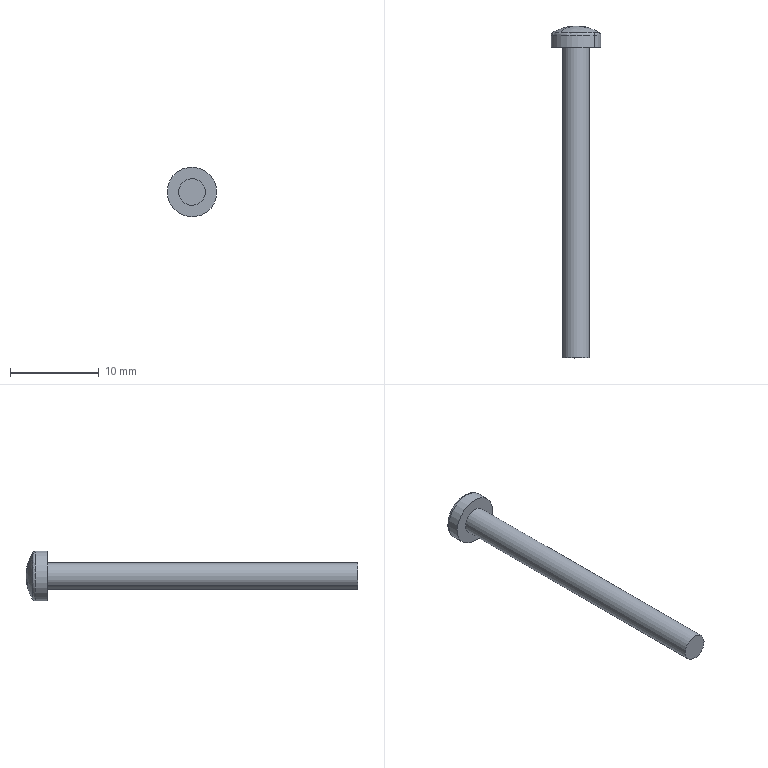Component | SolidWorks | pan cross head_am_pkg-12 | 1 solid | 23 faces | box 5.6 x 37.39 x 5.6 mm | volume 294 mm3 | plane 15 | cylinder 4 | torus 2 | sphere 2 | commonest cylinder face diameters 5.6 x2 3 x2
STEP:
#1=COLOUR_RGB('',0.7922,0.8196,0.9333);
#2=FILL_AREA_STYLE_COLOUR('',#1);
#3=FILL_AREA_STYLE('',(#2));
#4=SURFACE_STYLE_FILL_AREA(#3);
#5=SURFACE_SIDE_STYLE('',(#4));
#6=SURFACE_STYLE_USAGE(.BOTH.,#5);
#7=PRESENTATION_STYLE_ASSIGNMENT((#6));
#8=CARTESIAN_POINT('',(-1.144,1.16,0.966));
#9=VERTEX_POINT('',#8);
#10=CARTESIAN_POINT('',(-1.306,1.16,0.8157));
#11=VERTEX_POINT('',#10);
#12=CARTESIAN_POINT('',(-1.225,1.16,0.8908));
#13=DIRECTION('',(-0.,1.,-0.));
#14=DIRECTION('',(0.7319,0.,0.6814));
#15=AXIS2_PLACEMENT_3D('',#12,#13,#14);
#16=CIRCLE('',#15,0.1102);
#17=EDGE_CURVE('',#9,#11,#16,.T.);
#18=ORIENTED_EDGE('',*,*,#17,.T.);
#19=CARTESIAN_POINT('',(-1.301,1.171,0.82));
#20=VERTEX_POINT('',#19);
#21=CARTESIAN_POINT('',(-1.296,1.16,0.8247));
#22=DIRECTION('',(0.6814,0.,-0.7319));
#23=DIRECTION('',(-0.7319,0.,-0.6814));
#24=AXIS2_PLACEMENT_3D('',#21,#22,#23);
#25=CIRCLE('',#24,0.01323);
#26=EDGE_CURVE('',#11,#20,#25,.T.);
#27=ORIENTED_EDGE('',*,*,#26,.T.);
#28=CARTESIAN_POINT('',(-1.154,1.171,0.8147));
#29=VERTEX_POINT('',#28);
#30=CARTESIAN_POINT('',(-1.225,1.171,0.8908));
#31=DIRECTION('',(-0.,1.,-0.));
#32=DIRECTION('',(0.7319,0.,0.6814));
#33=AXIS2_PLACEMENT_3D('',#30,#31,#32);
#34=CIRCLE('',#33,0.104);
#35=EDGE_CURVE('',#29,#20,#34,.T.);
#36=ORIENTED_EDGE('',*,*,#35,.F.);
#37=CARTESIAN_POINT('',(-1.149,1.171,0.9617));
#38=VERTEX_POINT('',#37);
#39=CARTESIAN_POINT('',(-1.225,1.171,0.8908));
#40=DIRECTION('',(-0.,1.,-0.));
#41=DIRECTION('',(0.7319,0.,0.6814));
#42=AXIS2_PLACEMENT_3D('',#39,#40,#41);
#43=CIRCLE('',#42,0.104);
#44=EDGE_CURVE('',#38,#29,#43,.T.);
#45=ORIENTED_EDGE('',*,*,#44,.F.);
#46=CARTESIAN_POINT('',(-1.154,1.16,0.9569));
#47=DIRECTION('',(-0.6814,-0.,0.7319));
#48=DIRECTION('',(0.7319,0.,0.6814));
#49=AXIS2_PLACEMENT_3D('',#46,#47,#48);
#50=CIRCLE('',#49,0.01323);
#51=EDGE_CURVE('',#9,#38,#50,.T.);
#52=ORIENTED_EDGE('',*,*,#51,.F.);
#53=EDGE_LOOP('',(#18,#27,#36,#45,#52));
#54=FACE_OUTER_BOUND('',#53,.T.);
#55=CARTESIAN_POINT('',(-1.225,1.16,0.8908));
#56=DIRECTION('',(-0.,1.,-0.));
#57=DIRECTION('',(0.7319,0.,0.6814));
#58=AXIS2_PLACEMENT_3D('',#55,#56,#57);
#59=TOROIDAL_SURFACE('',#58,0.09701,0.01323);
#60=ADVANCED_FACE('',(#54),#59,.T.);
#61=CARTESIAN_POINT('',(-1.144,1.106,0.966));
#62=VERTEX_POINT('',#61);
#63=CARTESIAN_POINT('',(-1.306,1.106,0.8157));
#64=VERTEX_POINT('',#63);
#65=CARTESIAN_POINT('',(-1.225,1.106,0.8908));
#66=DIRECTION('',(-0.,1.,-0.));
#67=DIRECTION('',(0.7319,0.,0.6814));
#68=AXIS2_PLACEMENT_3D('',#65,#66,#67);
#69=CIRCLE('',#68,0.1102);
#70=EDGE_CURVE('',#62,#64,#69,.T.);
#71=ORIENTED_EDGE('',*,*,#70,.T.);
#72=CARTESIAN_POINT('',(-1.306,2.201,0.8157));
#73=DIRECTION('',(-0.,1.,-0.));
#74=VECTOR('',#73,39.37);
#75=LINE('',#72,#74);
#76=EDGE_CURVE('',#64,#11,#75,.T.);
#77=ORIENTED_EDGE('',*,*,#76,.T.);
#78=ORIENTED_EDGE('',*,*,#17,.F.);
#79=CARTESIAN_POINT('',(-1.144,2.201,0.966));
#80=DIRECTION('',(-0.,1.,-0.));
#81=VECTOR('',#80,39.37);
#82=LINE('',#79,#81);
#83=EDGE_CURVE('',#62,#9,#82,.T.);
#84=ORIENTED_EDGE('',*,*,#83,.F.);
#85=EDGE_LOOP('',(#71,#77,#78,#84));
#86=FACE_OUTER_BOUND('',#85,.T.);
#87=CARTESIAN_POINT('',(-1.225,2.201,0.8908));
#88=DIRECTION('',(-0.,1.,-0.));
#89=DIRECTION('',(0.7319,0.,0.6814));
#90=AXIS2_PLACEMENT_3D('',#87,#88,#89);
#91=CYLINDRICAL_SURFACE('',#90,0.1102);
#92=ADVANCED_FACE('',(#86),#91,.T.);
#93=CARTESIAN_POINT('',(-1.182,-0.2717,0.9311));
#94=VERTEX_POINT('',#93);
#95=CARTESIAN_POINT('',(-1.268,-0.2717,0.8506));
#96=VERTEX_POINT('',#95);
#97=CARTESIAN_POINT('',(-1.225,-0.2717,0.8908));
#98=DIRECTION('',(-0.,1.,-0.));
#99=DIRECTION('',(0.7319,0.,0.6814));
#100=AXIS2_PLACEMENT_3D('',#97,#98,#99);
#101=CIRCLE('',#100,0.05906);
#102=EDGE_CURVE('',#94,#96,#101,.T.);
#103=ORIENTED_EDGE('',*,*,#102,.T.);
#104=CARTESIAN_POINT('',(-1.268,1.106,0.8506));
#105=VERTEX_POINT('',#104);
#106=CARTESIAN_POINT('',(-1.268,2.201,0.8506));
#107=DIRECTION('',(-0.,1.,-0.));
#108=VECTOR('',#107,39.37);
#109=LINE('',#106,#108);
#110=EDGE_CURVE('',#96,#105,#109,.T.);
#111=ORIENTED_EDGE('',*,*,#110,.T.);
#112=CARTESIAN_POINT('',(-1.182,1.106,0.9311));
#113=VERTEX_POINT('',#112);
#114=CARTESIAN_POINT('',(-1.225,1.106,0.8908));
#115=DIRECTION('',(-0.,1.,-0.));
#116=DIRECTION('',(0.7319,0.,0.6814));
#117=AXIS2_PLACEMENT_3D('',#114,#115,#116);
#118=CIRCLE('',#117,0.05906);
#119=EDGE_CURVE('',#113,#105,#118,.T.);
#120=ORIENTED_EDGE('',*,*,#119,.F.);
#121=CARTESIAN_POINT('',(-1.182,2.201,0.9311));
#122=DIRECTION('',(-0.,1.,-0.));
#123=VECTOR('',#122,39.37);
#124=LINE('',#121,#123);
#125=EDGE_CURVE('',#94,#113,#124,.T.);
#126=ORIENTED_EDGE('',*,*,#125,.F.);
#127=EDGE_LOOP('',(#103,#111,#120,#126));
#128=FACE_OUTER_BOUND('',#127,.T.);
#129=CARTESIAN_POINT('',(-1.225,2.201,0.8908));
#130=DIRECTION('',(-0.,1.,-0.));
#131=DIRECTION('',(0.7319,0.,0.6814));
#132=AXIS2_PLACEMENT_3D('',#129,#130,#131);
#133=CYLINDRICAL_SURFACE('',#132,0.05906);
#134=ADVANCED_FACE('',(#128),#133,.T.);
#135=ORIENTED_EDGE('',*,*,#35,.T.);
#136=CARTESIAN_POINT('',(-1.296,1.171,0.967));
#137=VERTEX_POINT('',#136);
#138=CARTESIAN_POINT('',(-1.225,1.171,0.8908));
#139=DIRECTION('',(-0.,1.,-0.));
#140=DIRECTION('',(0.7319,0.,0.6814));
#141=AXIS2_PLACEMENT_3D('',#138,#139,#140);
#142=CIRCLE('',#141,0.104);
#143=EDGE_CURVE('',#20,#137,#142,.T.);
#144=ORIENTED_EDGE('',*,*,#143,.T.);
#145=CARTESIAN_POINT('',(-1.26,1.194,0.9286));
#146=VERTEX_POINT('',#145);
#147=CARTESIAN_POINT('',(-1.225,1.004,0.8908));
#148=DIRECTION('',(-0.7319,-0.,-0.6814));
#149=DIRECTION('',(-0.6814,0.,0.7319));
#150=AXIS2_PLACEMENT_3D('',#147,#148,#149);
#151=CIRCLE('',#150,0.1969);
#152=EDGE_CURVE('',#137,#146,#151,.T.);
#153=ORIENTED_EDGE('',*,*,#152,.T.);
#154=CARTESIAN_POINT('',(-1.267,1.194,0.9219));
#155=VERTEX_POINT('',#154);
#156=CARTESIAN_POINT('',(-1.19,1.038,0.8529));
#157=DIRECTION('',(-0.5674,-0.5538,0.6094));
#158=DIRECTION('',(0.3774,-0.8327,-0.4053));
#159=AXIS2_PLACEMENT_3D('',#156,#157,#158);
#160=CIRCLE('',#159,0.1867);
#161=EDGE_CURVE('',#146,#155,#160,.T.);
#162=ORIENTED_EDGE('',*,*,#161,.T.);
#163=CARTESIAN_POINT('',(-1.239,1.2,0.8914));
#164=VERTEX_POINT('',#163);
#165=CARTESIAN_POINT('',(-1.223,1.004,0.8928));
#166=DIRECTION('',(0.7303,0.06592,0.6799));
#167=DIRECTION('',(0.04824,-0.9978,0.04492));
#168=AXIS2_PLACEMENT_3D('',#165,#166,#167);
#169=CIRCLE('',#168,0.1968);
#170=EDGE_CURVE('',#164,#155,#169,.T.);
#171=ORIENTED_EDGE('',*,*,#170,.F.);
#172=CARTESIAN_POINT('',(-1.269,1.194,0.8629));
#173=VERTEX_POINT('',#172);
#174=CARTESIAN_POINT('',(-1.223,1.004,0.8888));
#175=DIRECTION('',(0.6799,0.06592,-0.7303));
#176=DIRECTION('',(-0.04492,0.9978,0.04824));
#177=AXIS2_PLACEMENT_3D('',#174,#175,#176);
#178=CIRCLE('',#177,0.1968);
#179=EDGE_CURVE('',#173,#164,#178,.T.);
#180=ORIENTED_EDGE('',*,*,#179,.F.);
#181=CARTESIAN_POINT('',(-1.256,1.194,0.8487));
#182=VERTEX_POINT('',#181);
#183=CARTESIAN_POINT('',(-1.187,1.038,0.9262));
#184=DIRECTION('',(-0.6094,-0.5538,-0.5674));
#185=DIRECTION('',(-0.4053,0.8327,-0.3774));
#186=AXIS2_PLACEMENT_3D('',#183,#184,#185);
#187=CIRCLE('',#186,0.1867);
#188=EDGE_CURVE('',#173,#182,#187,.T.);
#189=ORIENTED_EDGE('',*,*,#188,.T.);
#190=CARTESIAN_POINT('',(-1.225,1.2,0.8766));
#191=VERTEX_POINT('',#190);
#192=CARTESIAN_POINT('',(-1.227,1.004,0.8929));
#193=DIRECTION('',(-0.6799,0.06592,0.7303));
#194=DIRECTION('',(-0.04492,-0.9978,0.04824));
#195=AXIS2_PLACEMENT_3D('',#192,#193,#194);
#196=CIRCLE('',#195,0.1968);
#197=EDGE_CURVE('',#191,#182,#196,.T.);
#198=ORIENTED_EDGE('',*,*,#197,.F.);
#199=CARTESIAN_POINT('',(-1.197,1.194,0.8466));
#200=VERTEX_POINT('',#199);
#201=CARTESIAN_POINT('',(-1.223,1.004,0.8928));
#202=DIRECTION('',(0.7303,0.06592,0.6799));
#203=DIRECTION('',(0.04824,-0.9978,0.04492));
#204=AXIS2_PLACEMENT_3D('',#201,#202,#203);
#205=CIRCLE('',#204,0.1968);
#206=EDGE_CURVE('',#200,#191,#205,.T.);
#207=ORIENTED_EDGE('',*,*,#206,.F.);
#208=CARTESIAN_POINT('',(-1.19,1.194,0.8531));
#209=VERTEX_POINT('',#208);
#210=CARTESIAN_POINT('',(-1.26,1.038,0.9288));
#211=DIRECTION('',(0.5674,-0.5538,-0.6094));
#212=DIRECTION('',(0.3774,0.8327,-0.4053));
#213=AXIS2_PLACEMENT_3D('',#210,#211,#212);
#214=CIRCLE('',#213,0.1867);
#215=EDGE_CURVE('',#200,#209,#214,.T.);
#216=ORIENTED_EDGE('',*,*,#215,.T.);
#217=CARTESIAN_POINT('',(-1.225,1.004,0.8908));
#218=DIRECTION('',(0.7319,0.,0.6814));
#219=DIRECTION('',(0.6814,0.,-0.7319));
#220=AXIS2_PLACEMENT_3D('',#217,#218,#219);
#221=CIRCLE('',#220,0.1969);
#222=EDGE_CURVE('',#29,#209,#221,.T.);
#223=ORIENTED_EDGE('',*,*,#222,.F.);
#224=EDGE_LOOP('',(#135,#144,#153,#162,#171,#180,#189,#198,#207,#216,#223));
#225=FACE_OUTER_BOUND('',#224,.T.);
#226=CARTESIAN_POINT('',(-1.225,1.004,0.8908));
#227=DIRECTION('',(-0.7319,-0.,-0.6814));
#228=DIRECTION('',(0.6814,0.,-0.7319));
#229=AXIS2_PLACEMENT_3D('',#226,#227,#228);
#230=SPHERICAL_SURFACE('',#229,0.1969);
#231=ADVANCED_FACE('',(#225),#230,.T.);
#232=ORIENTED_EDGE('',*,*,#152,.F.);
#233=CARTESIAN_POINT('',(-1.225,1.171,0.8908));
#234=DIRECTION('',(-0.,1.,-0.));
#235=DIRECTION('',(0.7319,0.,0.6814));
#236=AXIS2_PLACEMENT_3D('',#233,#234,#235);
#237=CIRCLE('',#236,0.104);
#238=EDGE_CURVE('',#137,#38,#237,.T.);
#239=ORIENTED_EDGE('',*,*,#238,.T.);
#240=ORIENTED_EDGE('',*,*,#44,.T.);
#241=ORIENTED_EDGE('',*,*,#222,.T.);
#242=CARTESIAN_POINT('',(-1.183,1.194,0.8598));
#243=VERTEX_POINT('',#242);
#244=CARTESIAN_POINT('',(-1.26,1.038,0.9288));
#245=DIRECTION('',(0.5674,-0.5538,-0.6094));
#246=DIRECTION('',(0.3774,0.8327,-0.4053));
#247=AXIS2_PLACEMENT_3D('',#244,#245,#246);
#248=CIRCLE('',#247,0.1867);
#249=EDGE_CURVE('',#209,#243,#248,.T.);
#250=ORIENTED_EDGE('',*,*,#249,.T.);
#251=CARTESIAN_POINT('',(-1.211,1.2,0.8903));
#252=VERTEX_POINT('',#251);
#253=CARTESIAN_POINT('',(-1.227,1.004,0.8889));
#254=DIRECTION('',(-0.7303,0.06592,-0.6799));
#255=DIRECTION('',(0.04824,0.9978,0.04492));
#256=AXIS2_PLACEMENT_3D('',#253,#254,#255);
#257=CIRCLE('',#256,0.1968);
#258=EDGE_CURVE('',#252,#243,#257,.T.);
#259=ORIENTED_EDGE('',*,*,#258,.F.);
#260=CARTESIAN_POINT('',(-1.181,1.194,0.9188));
#261=VERTEX_POINT('',#260);
#262=CARTESIAN_POINT('',(-1.227,1.004,0.8929));
#263=DIRECTION('',(-0.6799,0.06592,0.7303));
#264=DIRECTION('',(-0.04492,-0.9978,0.04824));
#265=AXIS2_PLACEMENT_3D('',#262,#263,#264);
#266=CIRCLE('',#265,0.1968);
#267=EDGE_CURVE('',#261,#252,#266,.T.);
#268=ORIENTED_EDGE('',*,*,#267,.F.);
#269=CARTESIAN_POINT('',(-1.194,1.194,0.9329));
#270=VERTEX_POINT('',#269);
#271=CARTESIAN_POINT('',(-1.263,1.038,0.8555));
#272=DIRECTION('',(0.6094,-0.5538,0.5674));
#273=DIRECTION('',(-0.4053,-0.8327,-0.3774));
#274=AXIS2_PLACEMENT_3D('',#271,#272,#273);
#275=CIRCLE('',#274,0.1867);
#276=EDGE_CURVE('',#261,#270,#275,.T.);
#277=ORIENTED_EDGE('',*,*,#276,.T.);
#278=CARTESIAN_POINT('',(-1.224,1.2,0.9051));
#279=VERTEX_POINT('',#278);
#280=CARTESIAN_POINT('',(-1.223,1.004,0.8888));
#281=DIRECTION('',(0.6799,0.06592,-0.7303));
#282=DIRECTION('',(-0.04492,0.9978,0.04824));
#283=AXIS2_PLACEMENT_3D('',#280,#281,#282);
#284=CIRCLE('',#283,0.1968);
#285=EDGE_CURVE('',#279,#270,#284,.T.);
#286=ORIENTED_EDGE('',*,*,#285,.F.);
#287=CARTESIAN_POINT('',(-1.253,1.194,0.9351));
#288=VERTEX_POINT('',#287);
#289=CARTESIAN_POINT('',(-1.227,1.004,0.8889));
#290=DIRECTION('',(-0.7303,0.06592,-0.6799));
#291=DIRECTION('',(0.04824,0.9978,0.04492));
#292=AXIS2_PLACEMENT_3D('',#289,#290,#291);
#293=CIRCLE('',#292,0.1968);
#294=EDGE_CURVE('',#288,#279,#293,.T.);
#295=ORIENTED_EDGE('',*,*,#294,.F.);
#296=CARTESIAN_POINT('',(-1.19,1.038,0.8529));
#297=DIRECTION('',(-0.5674,-0.5538,0.6094));
#298=DIRECTION('',(0.3774,-0.8327,-0.4053));
#299=AXIS2_PLACEMENT_3D('',#296,#297,#298);
#300=CIRCLE('',#299,0.1867);
#301=EDGE_CURVE('',#288,#146,#300,.T.);
#302=ORIENTED_EDGE('',*,*,#301,.T.);
#303=EDGE_LOOP('',(#232,#239,#240,#241,#250,#259,#268,#277,#286,#295,#302));
#304=FACE_OUTER_BOUND('',#303,.T.);
#305=CARTESIAN_POINT('',(-1.225,1.004,0.8908));
#306=DIRECTION('',(-0.7319,-0.,-0.6814));
#307=DIRECTION('',(0.6814,0.,-0.7319));
#308=AXIS2_PLACEMENT_3D('',#305,#306,#307);
#309=SPHERICAL_SURFACE('',#308,0.1969);
#310=ADVANCED_FACE('',(#304),#309,.T.);
#311=ORIENTED_EDGE('',*,*,#206,.T.);
#312=CARTESIAN_POINT('',(-1.225,1.124,0.8837));
#313=VERTEX_POINT('',#312);
#314=CARTESIAN_POINT('',(-1.225,1.116,0.8844));
#315=DIRECTION('',(0.003322,-0.9957,0.09296));
#316=VECTOR('',#315,39.37);
#317=LINE('',#314,#316);
#318=EDGE_CURVE('',#191,#313,#317,.T.);
#319=ORIENTED_EDGE('',*,*,#318,.T.);
#320=CARTESIAN_POINT('',(-1.194,1.201,0.8429));
#321=DIRECTION('',(-0.3366,-0.8314,0.4421));
#322=VECTOR('',#321,39.37);
#323=LINE('',#320,#322);
#324=EDGE_CURVE('',#200,#313,#323,.T.);
#325=ORIENTED_EDGE('',*,*,#324,.F.);
#326=EDGE_LOOP('',(#311,#319,#325));
#327=FACE_OUTER_BOUND('',#326,.T.);
#328=CARTESIAN_POINT('',(-1.228,1.116,0.8877));
#329=DIRECTION('',(0.7303,0.06592,0.6799));
#330=DIRECTION('',(0.04824,-0.9978,0.04492));
#331=AXIS2_PLACEMENT_3D('',#328,#329,#330);
#332=PLANE('',#331);
#333=ADVANCED_FACE('',(#327),#332,.T.);
#334=CARTESIAN_POINT('',(-1.232,1.124,0.8911));
#335=VERTEX_POINT('',#334);
#336=CARTESIAN_POINT('',(-1.271,1.201,0.925));
#337=DIRECTION('',(0.417,-0.8314,-0.3673));
#338=VECTOR('',#337,39.37);
#339=LINE('',#336,#338);
#340=EDGE_CURVE('',#155,#335,#339,.T.);
#341=ORIENTED_EDGE('',*,*,#340,.T.);
#342=CARTESIAN_POINT('',(-1.231,1.116,0.8911));
#343=DIRECTION('',(-0.09296,0.9957,0.003322));
#344=VECTOR('',#343,39.37);
#345=LINE('',#342,#344);
#346=EDGE_CURVE('',#335,#164,#345,.T.);
#347=ORIENTED_EDGE('',*,*,#346,.T.);
#348=ORIENTED_EDGE('',*,*,#170,.T.);
#349=EDGE_LOOP('',(#341,#347,#348));
#350=FACE_OUTER_BOUND('',#349,.T.);
#351=CARTESIAN_POINT('',(-1.228,1.116,0.8877));
#352=DIRECTION('',(0.7303,0.06592,0.6799));
#353=DIRECTION('',(0.04824,-0.9978,0.04492));
#354=AXIS2_PLACEMENT_3D('',#351,#352,#353);
#355=PLANE('',#354);
#356=ADVANCED_FACE('',(#350),#355,.T.);
#357=CARTESIAN_POINT('',(-1.218,1.124,0.8906));
#358=VERTEX_POINT('',#357);
#359=CARTESIAN_POINT('',(-1.179,1.201,0.8567));
#360=DIRECTION('',(-0.417,-0.8314,0.3673));
#361=VECTOR('',#360,39.37);
#362=LINE('',#359,#361);
#363=EDGE_CURVE('',#243,#358,#362,.T.);
#364=ORIENTED_EDGE('',*,*,#363,.T.);
#365=CARTESIAN_POINT('',(-1.218,1.116,0.8906));
#366=DIRECTION('',(0.09296,0.9957,-0.003322));
#367=VECTOR('',#366,39.37);
#368=LINE('',#365,#367);
#369=EDGE_CURVE('',#358,#252,#368,.T.);
#370=ORIENTED_EDGE('',*,*,#369,.T.);
#371=ORIENTED_EDGE('',*,*,#258,.T.);
#372=EDGE_LOOP('',(#364,#370,#371));
#373=FACE_OUTER_BOUND('',#372,.T.);
#374=CARTESIAN_POINT('',(-1.222,1.116,0.894));
#375=DIRECTION('',(-0.7303,0.06592,-0.6799));
#376=DIRECTION('',(0.04824,0.9978,0.04492));
#377=AXIS2_PLACEMENT_3D('',#374,#375,#376);
#378=PLANE('',#377);
#379=ADVANCED_FACE('',(#373),#378,.T.);
#380=ORIENTED_EDGE('',*,*,#294,.T.);
#381=CARTESIAN_POINT('',(-1.225,1.124,0.898));
#382=VERTEX_POINT('',#381);
#383=CARTESIAN_POINT('',(-1.225,1.116,0.8973));
#384=DIRECTION('',(-0.003322,-0.9957,-0.09296));
#385=VECTOR('',#384,39.37);
#386=LINE('',#383,#385);
#387=EDGE_CURVE('',#279,#382,#386,.T.);
#388=ORIENTED_EDGE('',*,*,#387,.T.);
#389=CARTESIAN_POINT('',(-1.256,1.201,0.9388));
#390=DIRECTION('',(0.3366,-0.8314,-0.4421));
#391=VECTOR('',#390,39.37);
#392=LINE('',#389,#391);
#393=EDGE_CURVE('',#288,#382,#392,.T.);
#394=ORIENTED_EDGE('',*,*,#393,.F.);
#395=EDGE_LOOP('',(#380,#388,#394));
#396=FACE_OUTER_BOUND('',#395,.T.);
#397=CARTESIAN_POINT('',(-1.222,1.116,0.894));
#398=DIRECTION('',(-0.7303,0.06592,-0.6799));
#399=DIRECTION('',(0.04824,0.9978,0.04492));
#400=AXIS2_PLACEMENT_3D('',#397,#398,#399);
#401=PLANE('',#400);
#402=ADVANCED_FACE('',(#396),#401,.T.);
#403=ORIENTED_EDGE('',*,*,#110,.F.);
#404=CARTESIAN_POINT('',(-1.225,-0.2717,0.8908));
#405=DIRECTION('',(-0.,1.,-0.));
#406=DIRECTION('',(0.7319,0.,0.6814));
#407=AXIS2_PLACEMENT_3D('',#404,#405,#406);
#408=CIRCLE('',#407,0.05906);
#409=EDGE_CURVE('',#96,#94,#408,.T.);
#410=ORIENTED_EDGE('',*,*,#409,.T.);
#411=ORIENTED_EDGE('',*,*,#125,.T.);
#412=CARTESIAN_POINT('',(-1.225,1.106,0.8908));
#413=DIRECTION('',(-0.,1.,-0.));
#414=DIRECTION('',(0.7319,0.,0.6814));
#415=AXIS2_PLACEMENT_3D('',#412,#413,#414);
#416=CIRCLE('',#415,0.05906);
#417=EDGE_CURVE('',#105,#113,#416,.T.);
#418=ORIENTED_EDGE('',*,*,#417,.F.);
#419=EDGE_LOOP('',(#403,#410,#411,#418));
#420=FACE_OUTER_BOUND('',#419,.T.);
#421=CARTESIAN_POINT('',(-1.225,2.201,0.8908));
#422=DIRECTION('',(-0.,1.,-0.));
#423=DIRECTION('',(0.7319,0.,0.6814));
#424=AXIS2_PLACEMENT_3D('',#421,#422,#423);
#425=CYLINDRICAL_SURFACE('',#424,0.05906);
#426=ADVANCED_FACE('',(#420),#425,.T.);
#427=ORIENTED_EDGE('',*,*,#70,.F.);
#428=CARTESIAN_POINT('',(-1.225,1.106,0.8908));
#429=DIRECTION('',(-0.,1.,-0.));
#430=DIRECTION('',(0.7319,0.,0.6814));
#431=AXIS2_PLACEMENT_3D('',#428,#429,#430);
#432=CIRCLE('',#431,0.1102);
#433=EDGE_CURVE('',#64,#62,#432,.T.);
#434=ORIENTED_EDGE('',*,*,#433,.F.);
#435=EDGE_LOOP('',(#427,#434));
#436=FACE_OUTER_BOUND('',#435,.T.);
#437=ORIENTED_EDGE('',*,*,#119,.T.);
#438=ORIENTED_EDGE('',*,*,#417,.T.);
#439=EDGE_LOOP('',(#437,#438));
#440=FACE_BOUND('',#439,.T.);
#441=CARTESIAN_POINT('',(-1.185,1.106,0.8476));
#442=DIRECTION('',(-0.,1.,-0.));
#443=DIRECTION('',(0.7319,0.,0.6814));
#444=AXIS2_PLACEMENT_3D('',#441,#442,#443);
#445=PLANE('',#444);
#446=ADVANCED_FACE('',(#436,#440),#445,.F.);
#447=ORIENTED_EDGE('',*,*,#76,.F.);
#448=ORIENTED_EDGE('',*,*,#433,.T.);
#449=ORIENTED_EDGE('',*,*,#83,.T.);
#450=CARTESIAN_POINT('',(-1.225,1.16,0.8908));
#451=DIRECTION('',(-0.,1.,-0.));
#452=DIRECTION('',(0.7319,0.,0.6814));
#453=AXIS2_PLACEMENT_3D('',#450,#451,#452);
#454=CIRCLE('',#453,0.1102);
#455=EDGE_CURVE('',#11,#9,#454,.T.);
#456=ORIENTED_EDGE('',*,*,#455,.F.);
#457=EDGE_LOOP('',(#447,#448,#449,#456));
#458=FACE_OUTER_BOUND('',#457,.T.);
#459=CARTESIAN_POINT('',(-1.225,2.201,0.8908));
#460=DIRECTION('',(-0.,1.,-0.));
#461=DIRECTION('',(0.7319,0.,0.6814));
#462=AXIS2_PLACEMENT_3D('',#459,#460,#461);
#463=CYLINDRICAL_SURFACE('',#462,0.1102);
#464=ADVANCED_FACE('',(#458),#463,.T.);
#465=ORIENTED_EDGE('',*,*,#26,.F.);
#466=ORIENTED_EDGE('',*,*,#455,.T.);
#467=ORIENTED_EDGE('',*,*,#51,.T.);
#468=ORIENTED_EDGE('',*,*,#238,.F.);
#469=ORIENTED_EDGE('',*,*,#143,.F.);
#470=EDGE_LOOP('',(#465,#466,#467,#468,#469));
#471=FACE_OUTER_BOUND('',#470,.T.);
#472=CARTESIAN_POINT('',(-1.225,1.16,0.8908));
#473=DIRECTION('',(-0.,1.,-0.));
#474=DIRECTION('',(0.7319,0.,0.6814));
#475=AXIS2_PLACEMENT_3D('',#472,#473,#474);
#476=TOROIDAL_SURFACE('',#475,0.09701,0.01323);
#477=ADVANCED_FACE('',(#471),#476,.T.);
#478=ORIENTED_EDGE('',*,*,#102,.F.);
#479=ORIENTED_EDGE('',*,*,#409,.F.);
#480=EDGE_LOOP('',(#478,#479));
#481=FACE_OUTER_BOUND('',#480,.T.);
#482=CARTESIAN_POINT('',(-1.185,-0.2717,0.8476));
#483=DIRECTION('',(0.,-1.,0.));
#484=DIRECTION('',(-0.7319,-0.,-0.6814));
#485=AXIS2_PLACEMENT_3D('',#482,#483,#484);
#486=PLANE('',#485);
#487=ADVANCED_FACE('',(#481),#486,.T.);
#488=ORIENTED_EDGE('',*,*,#324,.T.);
#489=CARTESIAN_POINT('',(-1.218,1.124,0.8906));
#490=DIRECTION('',(-0.7319,-0.,-0.6814));
#491=VECTOR('',#490,39.37);
#492=LINE('',#489,#491);
#493=EDGE_CURVE('',#358,#313,#492,.T.);
#494=ORIENTED_EDGE('',*,*,#493,.F.);
#495=ORIENTED_EDGE('',*,*,#363,.F.);
#496=ORIENTED_EDGE('',*,*,#249,.F.);
#497=ORIENTED_EDGE('',*,*,#215,.F.);
#498=EDGE_LOOP('',(#488,#494,#495,#496,#497));
#499=FACE_OUTER_BOUND('',#498,.T.);
#500=CARTESIAN_POINT('',(-1.218,1.124,0.8906));
#501=DIRECTION('',(0.5674,-0.5538,-0.6094));
#502=DIRECTION('',(0.3774,0.8327,-0.4053));
#503=AXIS2_PLACEMENT_3D('',#500,#501,#502);
#504=PLANE('',#503);
#505=ADVANCED_FACE('',(#499),#504,.F.);
#506=ORIENTED_EDGE('',*,*,#393,.T.);
#507=CARTESIAN_POINT('',(-1.232,1.124,0.8911));
#508=DIRECTION('',(0.7319,0.,0.6814));
#509=VECTOR('',#508,39.37);
#510=LINE('',#507,#509);
#511=EDGE_CURVE('',#335,#382,#510,.T.);
#512=ORIENTED_EDGE('',*,*,#511,.F.);
#513=ORIENTED_EDGE('',*,*,#340,.F.);
#514=ORIENTED_EDGE('',*,*,#161,.F.);
#515=ORIENTED_EDGE('',*,*,#301,.F.);
#516=EDGE_LOOP('',(#506,#512,#513,#514,#515));
#517=FACE_OUTER_BOUND('',#516,.T.);
#518=CARTESIAN_POINT('',(-1.232,1.124,0.8911));
#519=DIRECTION('',(-0.5674,-0.5538,0.6094));
#520=DIRECTION('',(0.3774,-0.8327,-0.4053));
#521=AXIS2_PLACEMENT_3D('',#518,#519,#520);
#522=PLANE('',#521);
#523=ADVANCED_FACE('',(#517),#522,.F.);
#524=CARTESIAN_POINT('',(-1.232,1.124,0.8911));
#525=DIRECTION('',(0.6814,0.,-0.7319));
#526=VECTOR('',#525,39.37);
#527=LINE('',#524,#526);
#528=EDGE_CURVE('',#335,#313,#527,.T.);
#529=ORIENTED_EDGE('',*,*,#528,.F.);
#530=ORIENTED_EDGE('',*,*,#511,.T.);
#531=CARTESIAN_POINT('',(-1.218,1.124,0.8906));
#532=DIRECTION('',(-0.6814,-0.,0.7319));
#533=VECTOR('',#532,39.37);
#534=LINE('',#531,#533);
#535=EDGE_CURVE('',#358,#382,#534,.T.);
#536=ORIENTED_EDGE('',*,*,#535,.F.);
#537=ORIENTED_EDGE('',*,*,#493,.T.);
#538=EDGE_LOOP('',(#529,#530,#536,#537));
#539=FACE_OUTER_BOUND('',#538,.T.);
#540=CARTESIAN_POINT('',(-1.225,1.124,0.8837));
#541=DIRECTION('',(-0.,1.,-0.));
#542=DIRECTION('',(0.7319,0.,0.6814));
#543=AXIS2_PLACEMENT_3D('',#540,#541,#542);
#544=PLANE('',#543);
#545=ADVANCED_FACE('',(#539),#544,.T.);
#546=CARTESIAN_POINT('',(-1.273,1.201,0.86));
#547=DIRECTION('',(0.4421,-0.8314,0.3366));
#548=VECTOR('',#547,39.37);
#549=LINE('',#546,#548);
#550=EDGE_CURVE('',#173,#335,#549,.T.);
#551=ORIENTED_EDGE('',*,*,#550,.T.);
#552=ORIENTED_EDGE('',*,*,#528,.T.);
#553=CARTESIAN_POINT('',(-1.259,1.201,0.8452));
#554=DIRECTION('',(0.3673,-0.8314,0.417));
#555=VECTOR('',#554,39.37);
#556=LINE('',#553,#555);
#557=EDGE_CURVE('',#182,#313,#556,.T.);
#558=ORIENTED_EDGE('',*,*,#557,.F.);
#559=ORIENTED_EDGE('',*,*,#188,.F.);
#560=EDGE_LOOP('',(#551,#552,#558,#559));
#561=FACE_OUTER_BOUND('',#560,.T.);
#562=CARTESIAN_POINT('',(-1.225,1.124,0.8837));
#563=DIRECTION('',(-0.6094,-0.5538,-0.5674));
#564=DIRECTION('',(0.4053,-0.8327,0.3774));
#565=AXIS2_PLACEMENT_3D('',#562,#563,#564);
#566=PLANE('',#565);
#567=ADVANCED_FACE('',(#561),#566,.F.);
#568=ORIENTED_EDGE('',*,*,#179,.T.);
#569=ORIENTED_EDGE('',*,*,#346,.F.);
#570=ORIENTED_EDGE('',*,*,#550,.F.);
#571=EDGE_LOOP('',(#568,#569,#570));
#572=FACE_OUTER_BOUND('',#571,.T.);
#573=CARTESIAN_POINT('',(-1.228,1.116,0.8942));
#574=DIRECTION('',(0.6799,0.06592,-0.7303));
#575=DIRECTION('',(-0.04492,0.9978,0.04824));
#576=AXIS2_PLACEMENT_3D('',#573,#574,#575);
#577=PLANE('',#576);
#578=ADVANCED_FACE('',(#572),#577,.T.);
#579=ORIENTED_EDGE('',*,*,#197,.T.);
#580=ORIENTED_EDGE('',*,*,#557,.T.);
#581=ORIENTED_EDGE('',*,*,#318,.F.);
#582=EDGE_LOOP('',(#579,#580,#581));
#583=FACE_OUTER_BOUND('',#582,.T.);
#584=CARTESIAN_POINT('',(-1.222,1.116,0.8875));
#585=DIRECTION('',(-0.6799,0.06592,0.7303));
#586=DIRECTION('',(-0.04492,-0.9978,0.04824));
#587=AXIS2_PLACEMENT_3D('',#584,#585,#586);
#588=PLANE('',#587);
#589=ADVANCED_FACE('',(#583),#588,.T.);
#590=CARTESIAN_POINT('',(-1.177,1.201,0.9217));
#591=DIRECTION('',(-0.4421,-0.8314,-0.3366));
#592=VECTOR('',#591,39.37);
#593=LINE('',#590,#592);
#594=EDGE_CURVE('',#261,#358,#593,.T.);
#595=ORIENTED_EDGE('',*,*,#594,.T.);
#596=ORIENTED_EDGE('',*,*,#535,.T.);
#597=CARTESIAN_POINT('',(-1.191,1.201,0.9365));
#598=DIRECTION('',(-0.3673,-0.8314,-0.417));
#599=VECTOR('',#598,39.37);
#600=LINE('',#597,#599);
#601=EDGE_CURVE('',#270,#382,#600,.T.);
#602=ORIENTED_EDGE('',*,*,#601,.F.);
#603=ORIENTED_EDGE('',*,*,#276,.F.);
#604=EDGE_LOOP('',(#595,#596,#602,#603));
#605=FACE_OUTER_BOUND('',#604,.T.);
#606=CARTESIAN_POINT('',(-1.225,1.124,0.898));
#607=DIRECTION('',(0.6094,-0.5538,0.5674));
#608=DIRECTION('',(0.4053,0.8327,0.3774));
#609=AXIS2_PLACEMENT_3D('',#606,#607,#608);
#610=PLANE('',#609);
#611=ADVANCED_FACE('',(#605),#610,.F.);
#612=ORIENTED_EDGE('',*,*,#267,.T.);
#613=ORIENTED_EDGE('',*,*,#369,.F.);
#614=ORIENTED_EDGE('',*,*,#594,.F.);
#615=EDGE_LOOP('',(#612,#613,#614));
#616=FACE_OUTER_BOUND('',#615,.T.);
#617=CARTESIAN_POINT('',(-1.222,1.116,0.8875));
#618=DIRECTION('',(-0.6799,0.06592,0.7303));
#619=DIRECTION('',(-0.04492,-0.9978,0.04824));
#620=AXIS2_PLACEMENT_3D('',#617,#618,#619);
#621=PLANE('',#620);
#622=ADVANCED_FACE('',(#616),#621,.T.);
#623=ORIENTED_EDGE('',*,*,#285,.T.);
#624=ORIENTED_EDGE('',*,*,#601,.T.);
#625=ORIENTED_EDGE('',*,*,#387,.F.);
#626=EDGE_LOOP('',(#623,#624,#625));
#627=FACE_OUTER_BOUND('',#626,.T.);
#628=CARTESIAN_POINT('',(-1.228,1.116,0.8942));
#629=DIRECTION('',(0.6799,0.06592,-0.7303));
#630=DIRECTION('',(-0.04492,0.9978,0.04824));
#631=AXIS2_PLACEMENT_3D('',#628,#629,#630);
#632=PLANE('',#631);
#633=ADVANCED_FACE('',(#627),#632,.T.);
#634=CLOSED_SHELL('',(#60,#92,#134,#231,#310,#333,#356,#379,#402,#426,#446,#464,#477,#487,#505,#523,#545,#567,#578,#589,#611,#622,#633));
#635=MANIFOLD_SOLID_BREP('',#634);
#636=STYLED_ITEM('',(#7),#635);
#637=(LENGTH_UNIT()NAMED_UNIT(*)SI_UNIT($,.METRE.));
#638=LENGTH_MEASURE_WITH_UNIT(LENGTH_MEASURE(0.0254),#637);
#639=DIMENSIONAL_EXPONENTS(1.,0.,0.,0.,0.,0.,0.);
#640=(CONVERSION_BASED_UNIT('',#638)LENGTH_UNIT()NAMED_UNIT(#639));
#641=UNCERTAINTY_MEASURE_WITH_UNIT(LENGTH_MEASURE(0.00001),#640,'','');
#642=(NAMED_UNIT(*)PLANE_ANGLE_UNIT()SI_UNIT($,.RADIAN.));
#643=(NAMED_UNIT(*)SI_UNIT($,.STERADIAN.)SOLID_ANGLE_UNIT());
#644=(GEOMETRIC_REPRESENTATION_CONTEXT(3)GLOBAL_UNCERTAINTY_ASSIGNED_CONTEXT((#641))GLOBAL_UNIT_ASSIGNED_CONTEXT((#640,#642,#643))REPRESENTATION_CONTEXT('',''));
#645=MECHANICAL_DESIGN_GEOMETRIC_PRESENTATION_REPRESENTATION('',(#636),#644);
#646=PRESENTATION_LAYER_ASSIGNMENT('','',(#636));
#647=CARTESIAN_POINT('',(0.,0.,0.));
#648=DIRECTION('',(0.,0.,1.));
#649=DIRECTION('',(1.,0.,0.));
#650=AXIS2_PLACEMENT_3D('',#647,#648,#649);
#651=(LENGTH_UNIT()NAMED_UNIT(*)SI_UNIT($,.METRE.));
#652=LENGTH_MEASURE_WITH_UNIT(LENGTH_MEASURE(0.0254),#651);
#653=DIMENSIONAL_EXPONENTS(1.,0.,0.,0.,0.,0.,0.);
#654=(CONVERSION_BASED_UNIT('',#652)LENGTH_UNIT()NAMED_UNIT(#653));
#655=UNCERTAINTY_MEASURE_WITH_UNIT(LENGTH_MEASURE(0.00001),#654,'','');
#656=(NAMED_UNIT(*)PLANE_ANGLE_UNIT()SI_UNIT($,.RADIAN.));
#657=(NAMED_UNIT(*)SI_UNIT($,.STERADIAN.)SOLID_ANGLE_UNIT());
#658=(GEOMETRIC_REPRESENTATION_CONTEXT(3)GLOBAL_UNCERTAINTY_ASSIGNED_CONTEXT((#655))GLOBAL_UNIT_ASSIGNED_CONTEXT((#654,#656,#657))REPRESENTATION_CONTEXT('',''));
#659=ADVANCED_BREP_SHAPE_REPRESENTATION('',(#635,#650),#658);